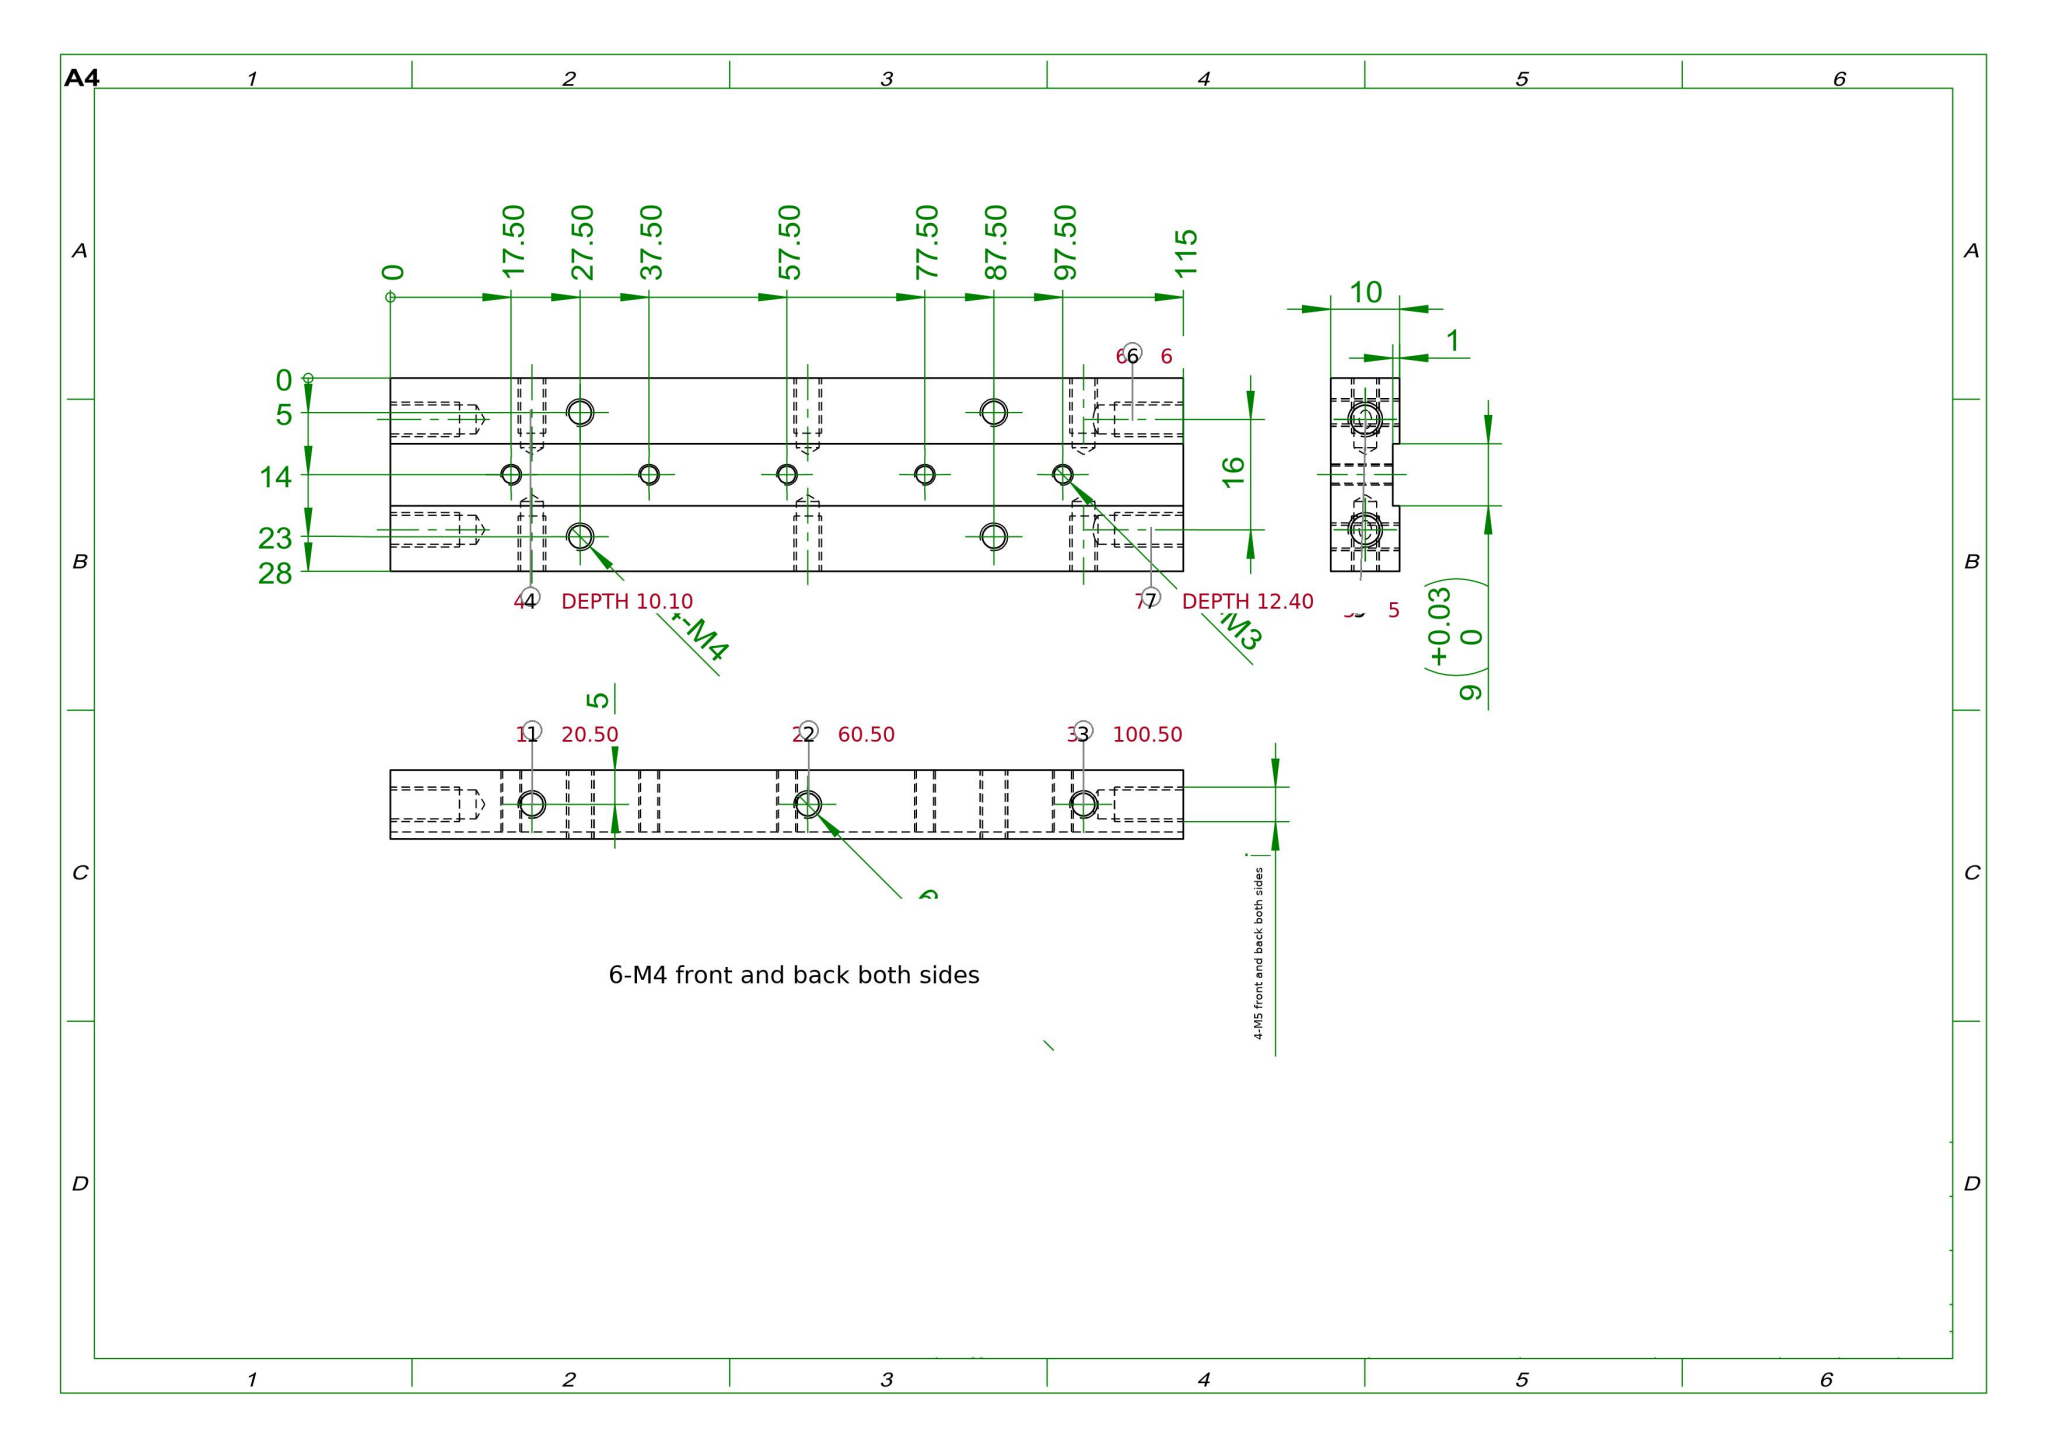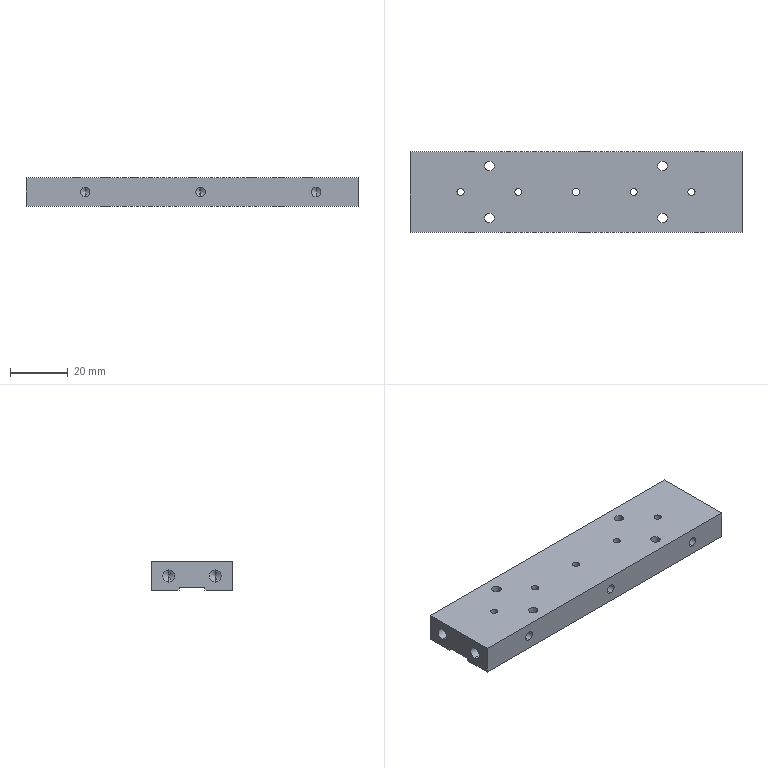Part | SolidWorks | mm | 1 solid | 68 faces | box 115 x 28 x 10 mm | volume 29358 mm3 | cylinder 38 | cone 20 | plane 10 | commonest cylinder face diameters 3.3 x20 2.5 x10 4.2 x8
build123d program:
from build123d import *

# Parameters (mm, degrees)
SKETCH1_W                  = 115
SKETCH1_H                  = 28
BOSS_EXTRUDE1_DEPTH        = 10
SKETCH2_W                  = 2
SKETCH2_H                  = 9
CUT_EXTRUDE1_DEPTH         = 117.28
M5_TAPPED_HOLE1_D          = 4.2
M5_TAPPED_HOLE1_DEPTH      = 12.4
M5_TAPPED_HOLE1_TIP        = 1.262
M5_TAPPED_HOLE2_D          = 4.2
M5_TAPPED_HOLE2_DEPTH      = 12.4
M5_TAPPED_HOLE2_TIP        = 1.262
M4_TAPPED_HOLE1_AT_2_COUNT = 2
M4_TAPPED_HOLE1_AT_2_PITCH = 40
M4_TAPPED_HOLE1_AT_3_COUNT = 2
M4_TAPPED_HOLE1_AT_3_PITCH = 80
M3_TAPPED_HOLE1_D          = 2.5
M4_TAPPED_HOLE2_D          = 3.3


with BuildPart() as part:
    # Sketch1 → Boss-Extrude1 (new body)
    with BuildSketch(Plane.XY):
        Rectangle(SKETCH1_W, SKETCH1_H)
    extrude(amount=BOSS_EXTRUDE1_DEPTH)

    # Sketch2 → Cut-Extrude1 (cut, through all)
    with BuildSketch(Plane.ZY.offset(57.5)):
        Rectangle(SKETCH2_W, SKETCH2_H)
    extrude(amount=-CUT_EXTRUDE1_DEPTH, mode=Mode.SUBTRACT)

    # M5 Tapped Hole1
    with Locations(Plane(origin=(57.5, 0, 0), x_dir=(0, 0, -1), z_dir=(1, 0, 0))):
        with Locations((-5, 8), (-5, -8)):
            Hole(M5_TAPPED_HOLE1_D / 2, depth=M5_TAPPED_HOLE1_DEPTH)
            with Locations((0, 0, -(M5_TAPPED_HOLE1_DEPTH + M5_TAPPED_HOLE1_TIP / 2))):  # 118° drill point
                Cone(0, M5_TAPPED_HOLE1_D / 2, M5_TAPPED_HOLE1_TIP, mode=Mode.SUBTRACT)

    # M5 Tapped Hole2
    with Locations(Plane.ZY.offset(57.5)):
        with Locations((5, -8), (5, 8)):
            Hole(M5_TAPPED_HOLE2_D / 2, depth=M5_TAPPED_HOLE2_DEPTH)
            with Locations((0, 0, -(M5_TAPPED_HOLE2_DEPTH + M5_TAPPED_HOLE2_TIP / 2))):  # 118° drill point
                Cone(0, M5_TAPPED_HOLE2_D / 2, M5_TAPPED_HOLE2_TIP, mode=Mode.SUBTRACT)

    # Sketch8 → M4 Tapped Hole1 (revolve, cut)
    with BuildSketch(Plane(origin=(43, -14, 5), x_dir=(0, 0, -1), z_dir=(1, 0, 0))):
        Polygon((0, 0), (0, 11.091), (1.65, 10.1), (1.65, 0), align=None)
    m4_tapped_hole1 = revolve(axis=Axis((43, -20.35, 5), (0, 1, 0)), mode=Mode.SUBTRACT)

    # M4 Tapped Hole1 at 2: M4 Tapped Hole1 ×2
    with Locations(*[(-i * M4_TAPPED_HOLE1_AT_2_PITCH, 0, 0) for i in range(1, M4_TAPPED_HOLE1_AT_2_COUNT)]):
        add(m4_tapped_hole1, mode=Mode.SUBTRACT)

    # M4 Tapped Hole1 at 3: M4 Tapped Hole1 ×2
    with Locations(*[(-i * M4_TAPPED_HOLE1_AT_3_PITCH, 0, 0) for i in range(1, M4_TAPPED_HOLE1_AT_3_COUNT)]):
        add(m4_tapped_hole1, mode=Mode.SUBTRACT)

    # Mirror1: M4 Tapped Hole1 across plane
    add(m4_tapped_hole1.mirror(Plane.ZX), mode=Mode.SUBTRACT)

    # Mirror1 copy 1 sketch → Mirror1 copy 1 (revolve, cut)
    with BuildSketch(Plane(origin=(3, 14, 5), x_dir=(0, 0, -1), z_dir=(1, 0, 0))):
        Polygon((0, 0), (0, -11.091), (1.65, -10.1), (1.65, 0), align=None)
    revolve(axis=Axis((3, 20.35, 5), (0, 1, 0)), mode=Mode.SUBTRACT)

    # Mirror1 copy 2 sketch → Mirror1 copy 2 (revolve, cut)
    with BuildSketch(Plane(origin=(-37, 14, 5), x_dir=(0, 0, -1), z_dir=(1, 0, 0))):
        Polygon((0, 0), (0, -11.091), (1.65, -10.1), (1.65, 0), align=None)
    revolve(axis=Axis((-37, 20.35, 5), (0, 1, 0)), mode=Mode.SUBTRACT)

    # M3 Tapped Hole1 (through all)
    with Locations(Plane(origin=(0, 0, 1), x_dir=(-1, 0, 0), z_dir=(0, 0, -1))):
        with Locations((-40, 0), (-20, 0), (0, 0), (20, 0), (40, 0)):
            Hole(M3_TAPPED_HOLE1_D / 2)

    # M4 Tapped Hole2 (through all)
    with Locations(Plane(origin=(0, 0, 0), x_dir=(-1, 0, 0), z_dir=(0, 0, -1))):
        with Locations((-30, 9), (30, 9), (30, -9), (-30, -9)):
            Hole(M4_TAPPED_HOLE2_D / 2)


solid = part.part